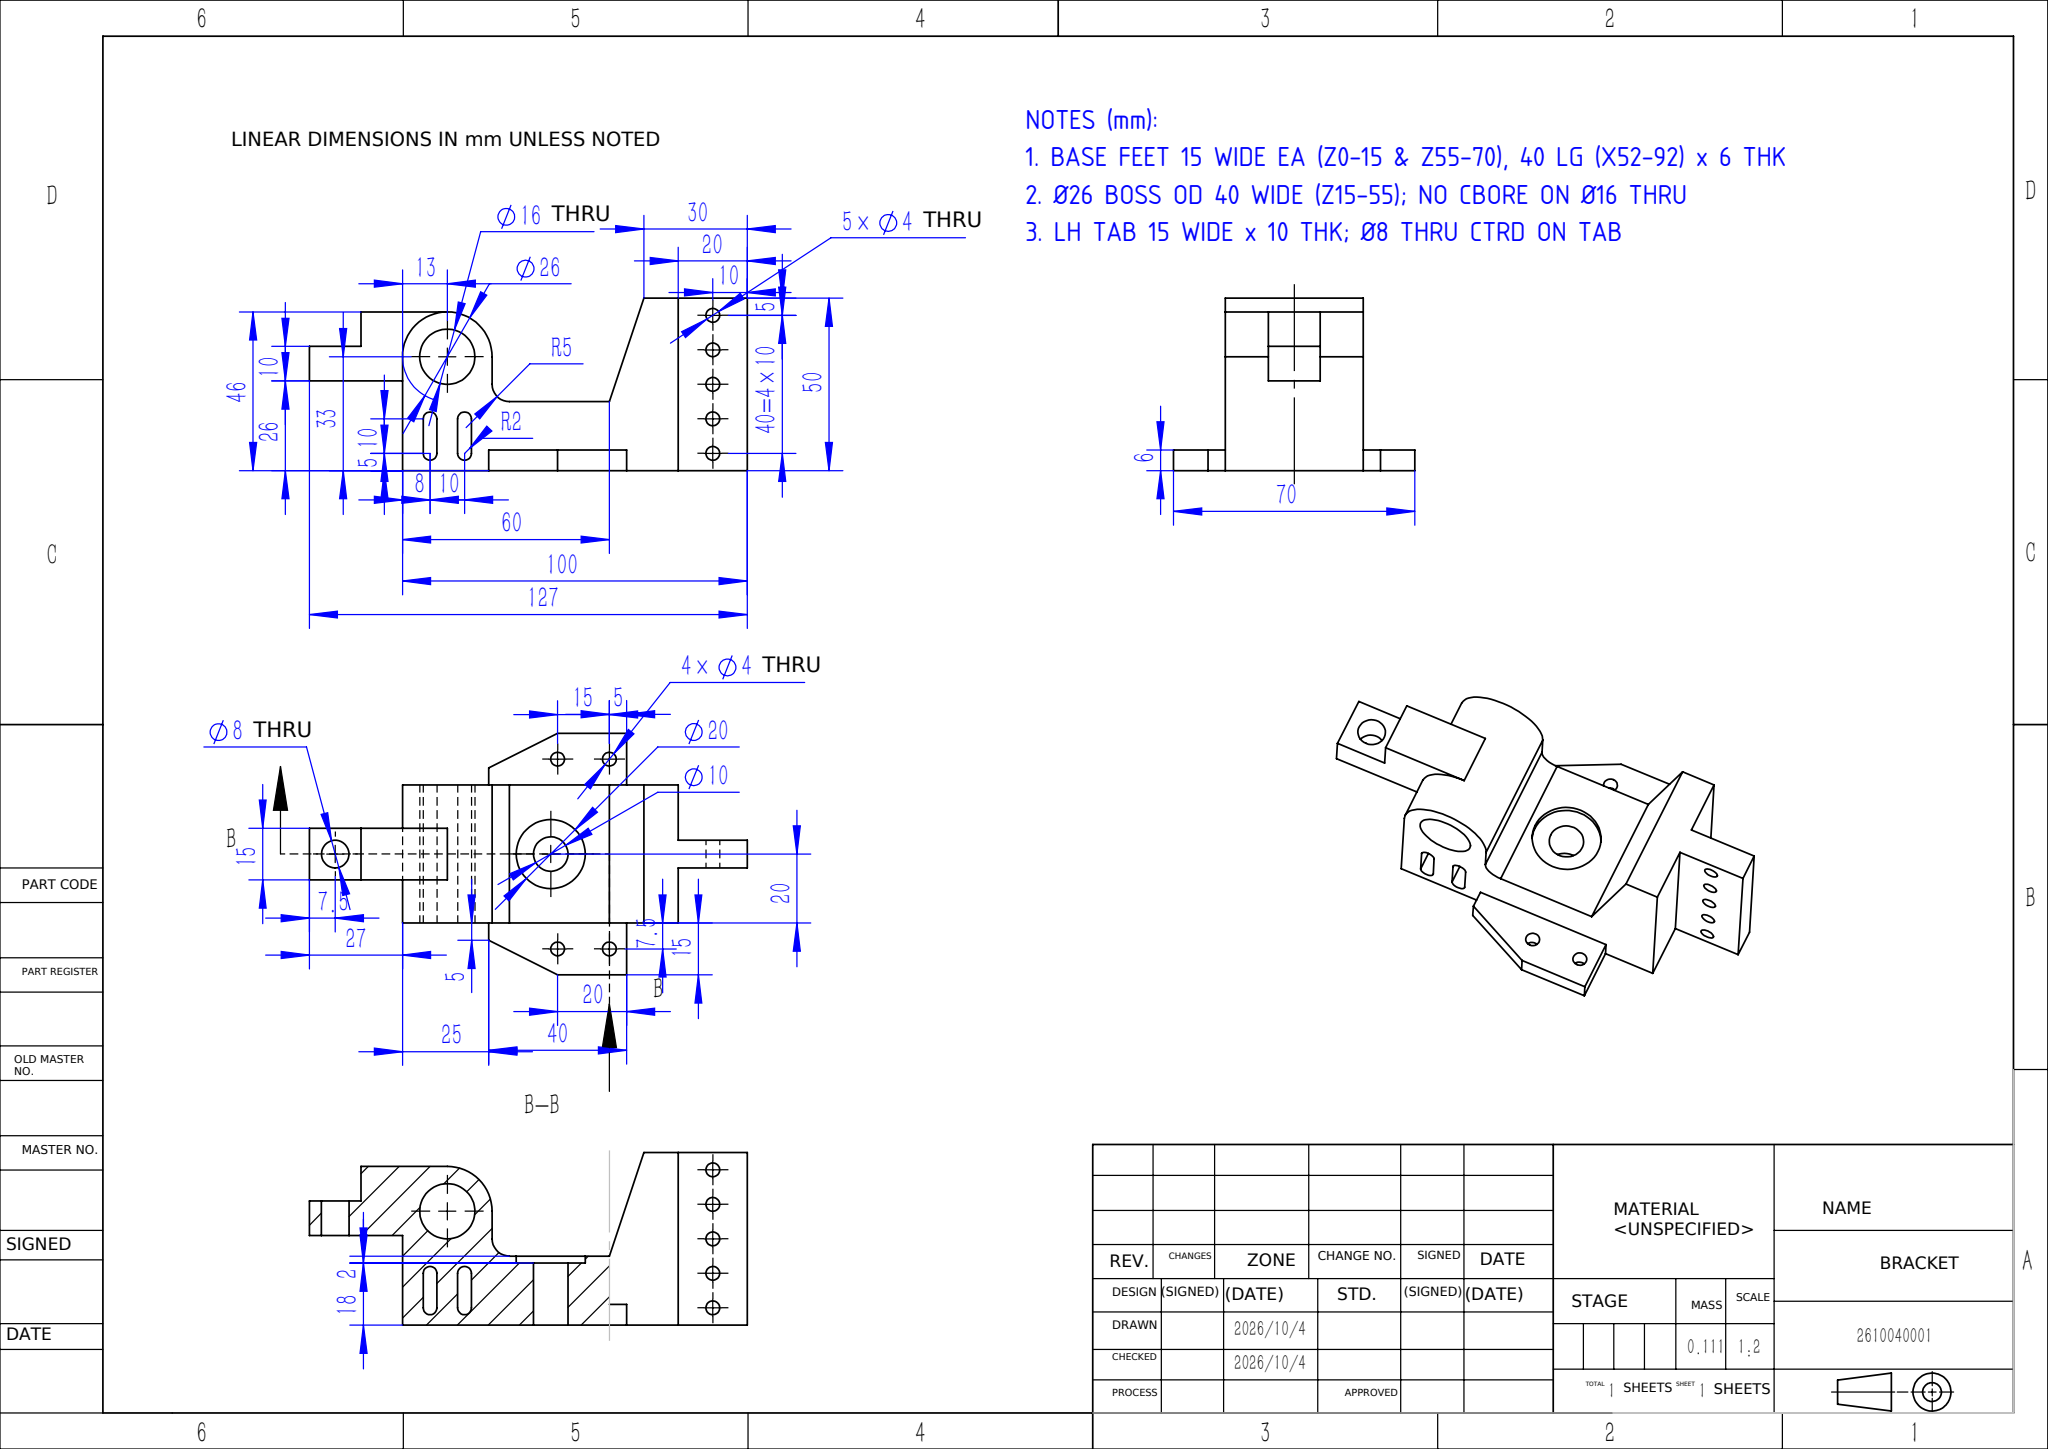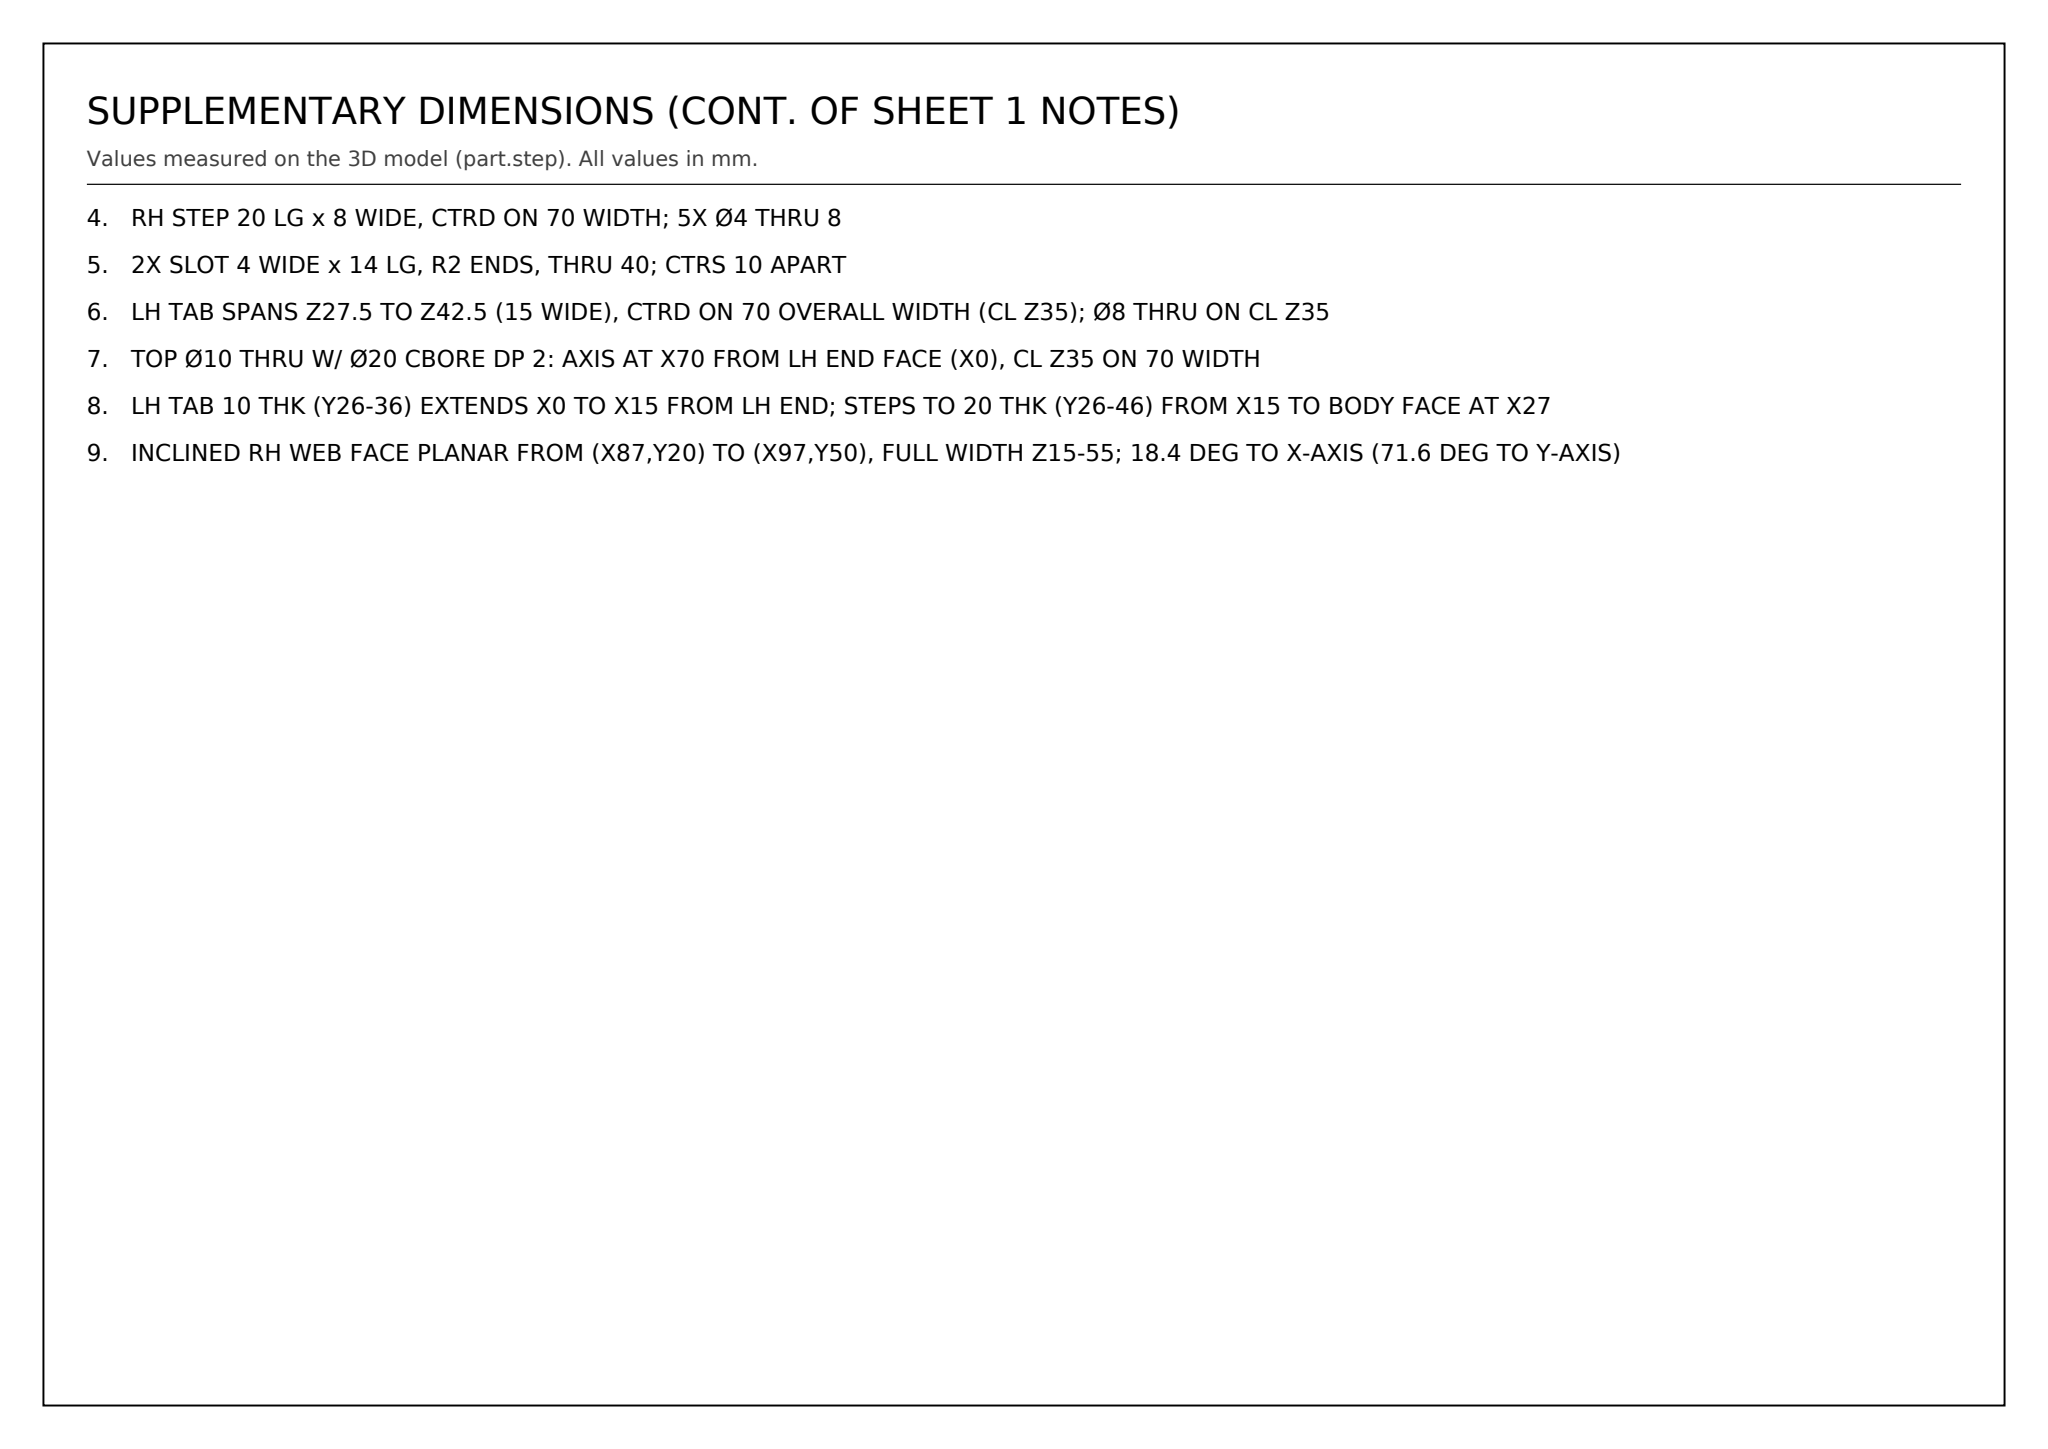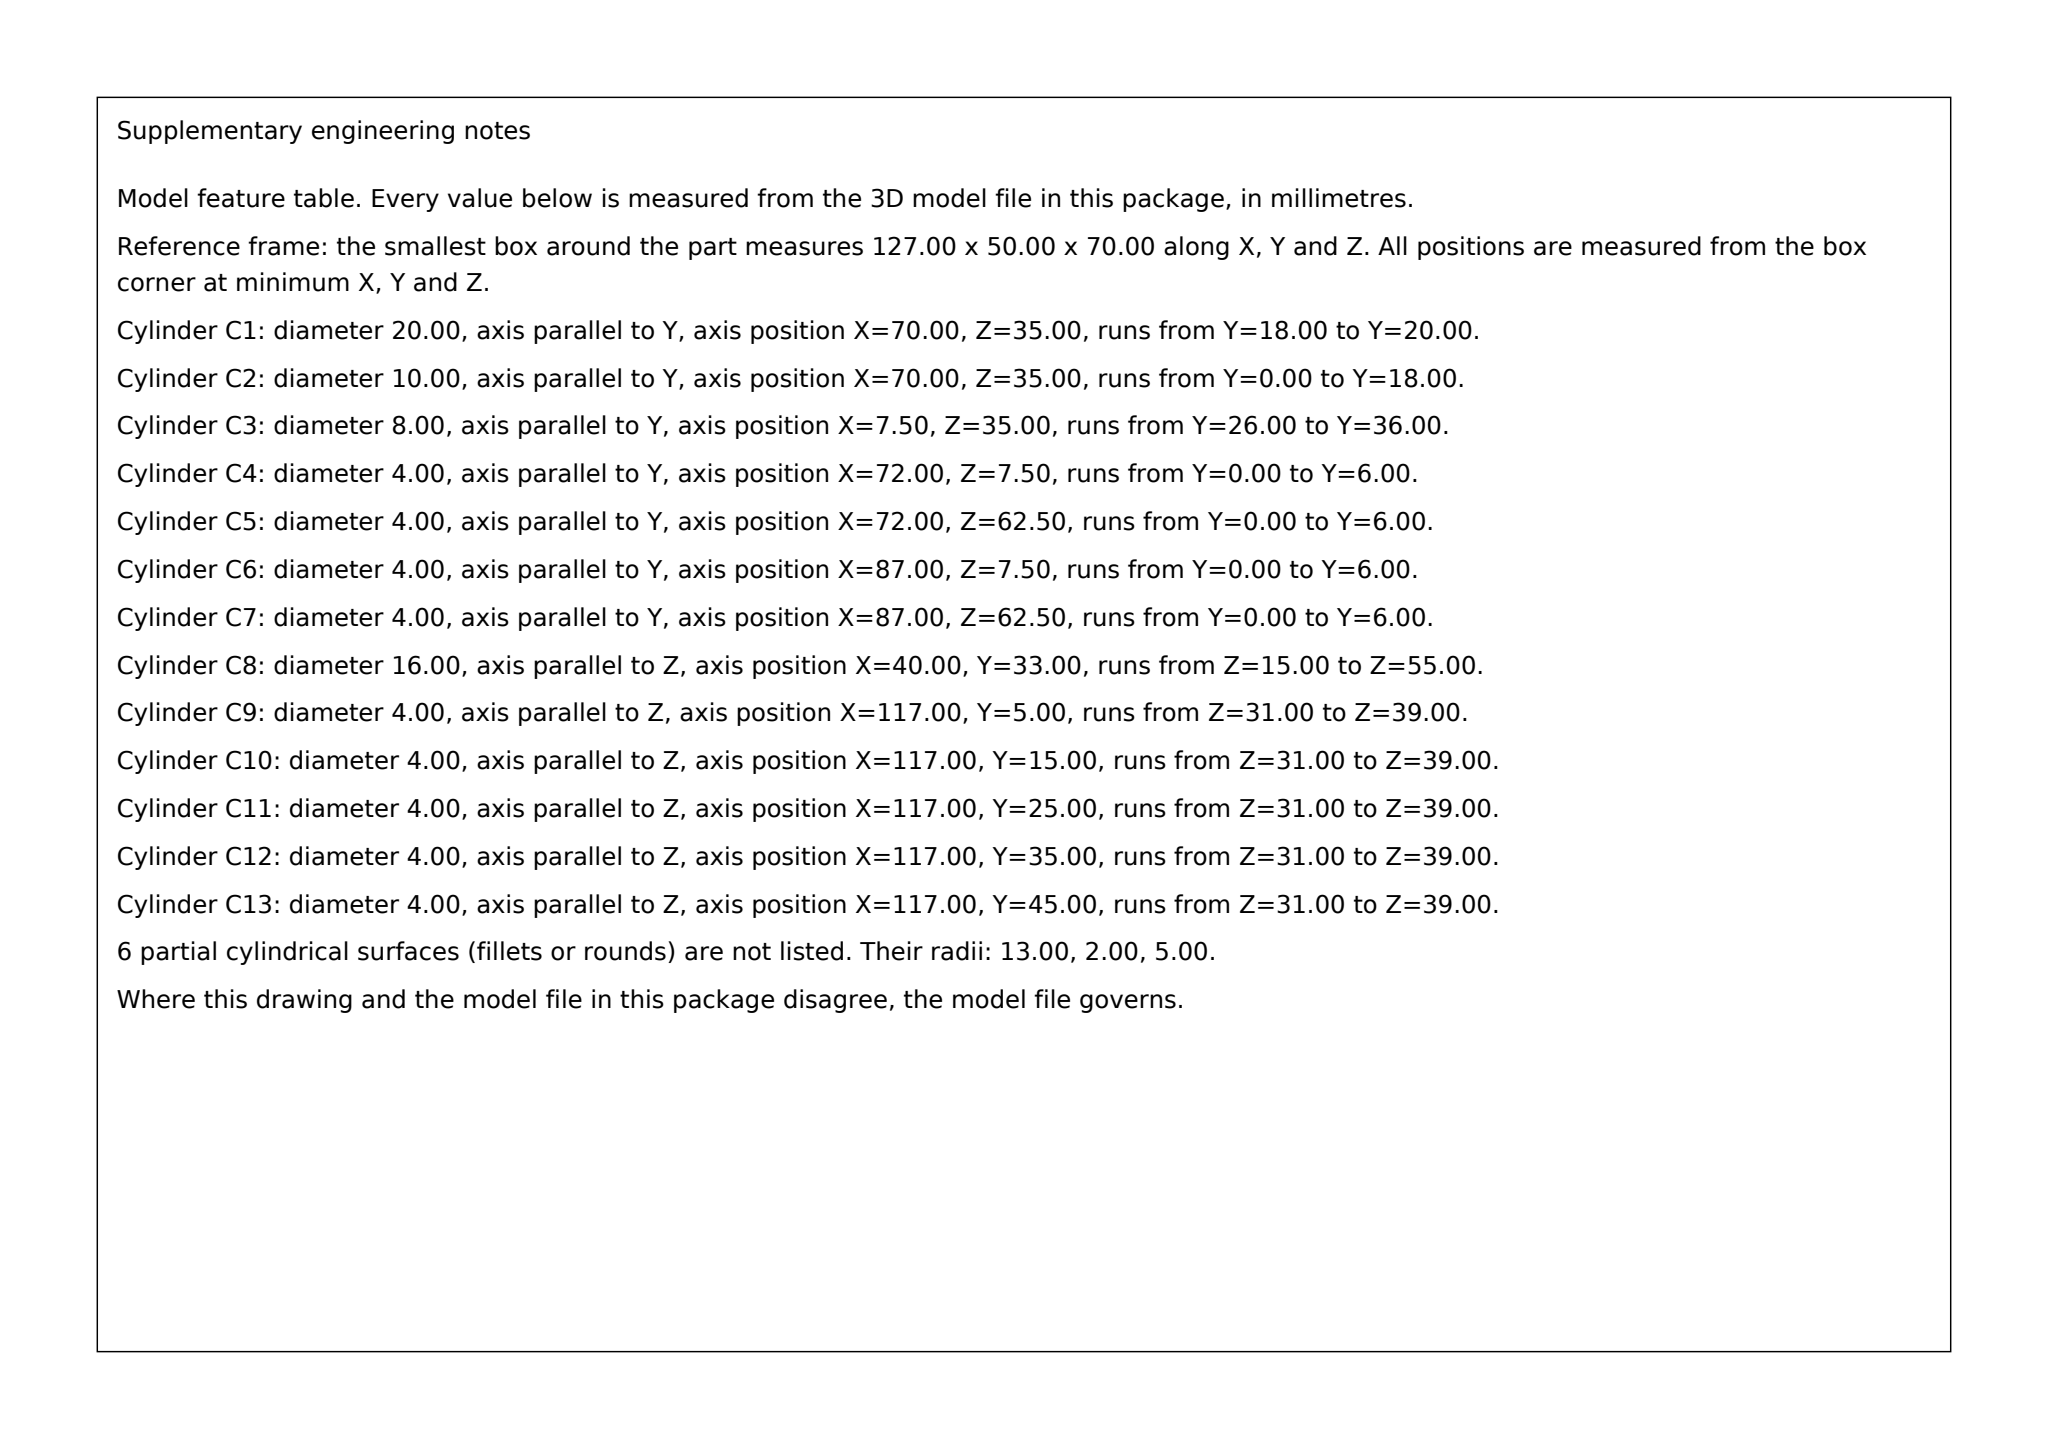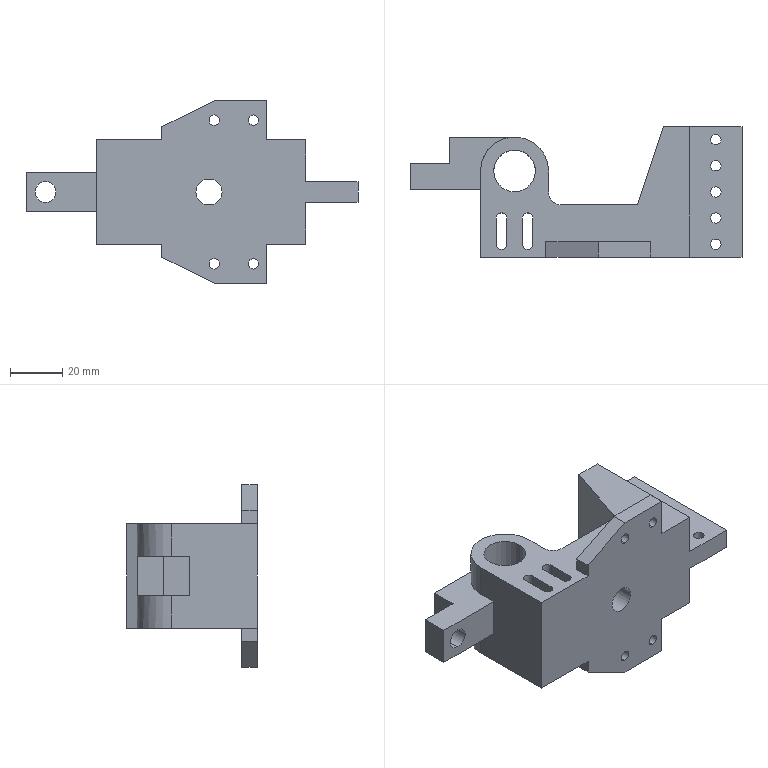Part | SolidWorks | mm | 1 solid | 67 faces | box 127 x 50 x 70 mm | volume 111150 mm3 | plane 35 | cylinder 32 | commonest cylinder face diameters 4 x22 10 x3 8 x2 20 x2 16 x2 26 x1
Drawing notes:
BASE FEET 15 WIDE EA (Z0-15 & Z55-70), 40 LG (X52-92) x 6 THK | from the solid: z-planes 0,15,55,70; x-planes 52 & 92; y-plane 6; dia4 axis y at z7.5 & z62.5 len 6
Ø26 BOSS OD 40 WIDE (Z15-55); NO CBORE ON Ø16 THRU | from the solid: Cyl Ø26 axis z at (40,33) len 40, z planes 15 & 55; Ø16 same axis len 40 thru, no intermediate z face
LH TAB 15 WIDE x 10 THK; Ø8 THRU CTRD ON TAB | from the solid: x-planes 0,15,27; z-planes 27.5/42.5; dia8 axis y at (7.5,35) len 10
RH STEP 20 LG x 8 WIDE, CTRD ON 70 WIDTH; 5X Ø4 THRU 8 | from the solid: x-planes 107 & 127; z-planes 31 & 39; 5X dia4 axis z at x117 len 8
2X SLOT 4 WIDE x 14 LG, R2 ENDS, THRU 40; CTRS 10 APART | from the solid: dia4 axis z at (35,5),(35,15),(45,5),(45,15) len 40 -> 4 wide, 14 OAL
LH TAB SPANS Z27.5 TO Z42.5 (15 WIDE), CTRD ON 70 OVERALL WIDTH (CL Z35); Ø8 THRU ON CL Z35 | from the solid: axis_planes x=0.0 extent z [27.5,42.5]; hole/bore dia 8.0 axis y at [7.5, null, 35.0] from 26.0 to 36.0
TOP Ø10 THRU W/ Ø20 CBORE DP 2: AXIS AT X70 FROM LH END FACE (X0), CL Z35 ON 70 WIDTH | from the solid: Ø10 bore, axis y at (x70, z35), from y0 to y18; Ø20 bore same axis from y18 to y20 (entry face y=20, cbore dp 2). The Ø10 reaches the bottom face y=0 (y=0 plane area 4231 only balances with the Ø10 opening), so the Ø10 is THRU the 20 thk section, not blind.
LH TAB 10 THK (Y26-36) EXTENDS X0 TO X15 FROM LH END; STEPS TO 20 THK (Y26-46) FROM X15 TO BODY FACE AT X27 | from the solid: axis_planes: y=36 over x[0,15] z[27.5,42.5]; y=46 over x[15,40] z[27.5,42.5]; x=15 over y[36,46]; x=27 over y[0,33]
INCLINED RH WEB FACE PLANAR FROM (X87,Y20) TO (X97,Y50), FULL WIDTH Z15-55; 18.4 DEG TO X-AXIS (71.6 DEG TO Y-AXIS) | from the solid: inclined_planes: angle_to_xyz_axes [18.4, 71.6, 90.0], bbox_from [87,20,15], size [10,30,40]
build123d program:
from build123d import *

# Parameters (mm, degrees)
BOSS_EXTRUDE1_DEPTH = 20
SKETCH2_W           = 20
SKETCH2_H           = 16
CUT_EXTRUDE1_DEPTH  = 114.578
SKETCH3_W           = 40
SKETCH3_H           = 15
BOSS_EXTRUDE2_DEPTH = 20
SKETCH4_W           = 15
SKETCH4_H           = 15
CUT_EXTRUDE2_DEPTH  = 10
BOSS_EXTRUDE3_DEPTH = 6
SKETCH6_R           = 8
CUT_EXTRUDE3_DEPTH  = 119.004
SKETCH7_R           = 10
CUT_EXTRUDE4_DEPTH  = 2
SKETCH8_R           = 5
CUT_EXTRUDE5_DEPTH  = 111.675
SKETCH9_R           = 2
CUT_EXTRUDE6_DEPTH  = 112.45
FILLET1_R           = 5
SKETCH10_R          = 4
CUT_EXTRUDE7_DEPTH  = 112.897
SKETCH11_R          = 2
CUT_EXTRUDE8_DEPTH  = 115.721
CUT_EXTRUDE9_DEPTH  = 119.004


with BuildPart() as part:
    # Sketch1 → Boss-Extrude1 (new, symmetric)
    with BuildSketch(Plane.XY):
        with BuildLine():
            Line((0, 0), (0, -20))
            Line((0, -20), (100, -20))
            Line((100, -20), (100, 30))
            Line((100, 30), (70, 30))
            Line((70, 30), (60, 0))
            Line((60, 0), (26, 0))
            Line((26, 0), (26, 13))
            ThreePointArc((26, 13), (13, 26), (0, 13))
            Line((0, 13), (0, 0))
        make_face()
    extrude(amount=BOSS_EXTRUDE1_DEPTH, both=True)

    # Sketch2 → Cut-Extrude1 (cut, through all)
    with BuildSketch(Plane(origin=(0, 30, 0), x_dir=(1, 0, 0), z_dir=(0, 1, 0))):
        with Locations((90, 12)):
            Rectangle(SKETCH2_W, SKETCH2_H)
        with Locations((90, -12)):
            Rectangle(SKETCH2_W, SKETCH2_H)
    extrude(amount=-CUT_EXTRUDE1_DEPTH, mode=Mode.SUBTRACT)

    # Sketch3 → Boss-Extrude2 (add)
    with BuildSketch(Plane(origin=(0, 26, 0), x_dir=(-1, 0, 0), z_dir=(0, -1, 0))):
        with Locations((7, 0)):
            Rectangle(SKETCH3_W, SKETCH3_H)
    extrude(amount=BOSS_EXTRUDE2_DEPTH)

    # Sketch4 → Cut-Extrude2 (cut)
    with BuildSketch(Plane(origin=(0, 26, 0), x_dir=(1, 0, 0), z_dir=(0, 1, 0))):
        with Locations((-19.5, 0)):
            Rectangle(SKETCH4_W, SKETCH4_H)
    extrude(amount=-CUT_EXTRUDE2_DEPTH, mode=Mode.SUBTRACT)

    # Sketch5 → Boss-Extrude3 (add)
    with BuildSketch(Plane.XZ.offset(20)):
        Polygon((65, 20), (65, 35), (45, 35), (25, 25), (25, 20), align=None)
        Polygon((25, -25), (25, -20), (65, -20), (65, -35), (45, -35), align=None)
    extrude(amount=-BOSS_EXTRUDE3_DEPTH)

    # Sketch6 → Cut-Extrude3 (cut, through all)
    with BuildSketch(Plane.XY.offset(20)):
        with Locations((13, 13)):
            Circle(SKETCH6_R)
    extrude(amount=-CUT_EXTRUDE3_DEPTH, mode=Mode.SUBTRACT)

    # Sketch7 → Cut-Extrude4 (cut)
    with BuildSketch(Plane(origin=(0, 0, 0), x_dir=(1, 0, 0), z_dir=(0, 1, 0))):
        with Locations(Location((43, 0, 0), (0, 0, 180))):
            Circle(SKETCH7_R)
    extrude(amount=-CUT_EXTRUDE4_DEPTH, mode=Mode.SUBTRACT)

    # Sketch8 → Cut-Extrude5 (cut, through all)
    with BuildSketch(Plane(origin=(0, -2, 0), x_dir=(1, 0, 0), z_dir=(0, 1, 0))):
        with Locations(Location((43, 0, 0), (0, 0, 180))):
            Circle(SKETCH8_R)
    extrude(amount=-CUT_EXTRUDE5_DEPTH, mode=Mode.SUBTRACT)

    # Sketch9 → Cut-Extrude6 (cut, through all)
    with BuildSketch(Plane.XY.offset(4)):
        with Locations((90, 25)):
            Circle(SKETCH9_R)
        with Locations((90, 15)):
            Circle(SKETCH9_R)
        with Locations((90, 5)):
            Circle(SKETCH9_R)
        with Locations((90, -5)):
            Circle(SKETCH9_R)
        with Locations((90, -15)):
            Circle(SKETCH9_R)
    extrude(amount=-CUT_EXTRUDE6_DEPTH, mode=Mode.SUBTRACT)

    # Fillet1
    fillet1_edges = [part.edges().sort_by_distance(p)[0] for p in [
        (26, 0, 0),
    ]]
    fillet(fillet1_edges, radius=FILLET1_R)

    # Sketch10 → Cut-Extrude7 (cut, through all)
    with BuildSketch(Plane(origin=(0, 16, 0), x_dir=(1, 0, 0), z_dir=(0, 1, 0))):
        with Locations(Location((-19.5, 0, 0), (0, 0, 270))):
            Circle(SKETCH10_R)
    extrude(amount=-CUT_EXTRUDE7_DEPTH, mode=Mode.SUBTRACT)

    # Sketch11 → Cut-Extrude8 (cut, through all)
    with BuildSketch(Plane(origin=(0, -14, 0), x_dir=(1, 0, 0), z_dir=(0, 1, 0))):
        with Locations(Location((60, -27.5, 0), (0, 0, 270))):
            Circle(SKETCH11_R)
        with Locations(Location((45, -27.5, 0), (0, 0, 270))):
            Circle(SKETCH11_R)
        with Locations(Location((60, 27.5, 0), (0, 0, 90))):
            Circle(SKETCH11_R)
        with Locations(Location((45, 27.5, 0), (0, 0, 90))):
            Circle(SKETCH11_R)
    extrude(amount=-CUT_EXTRUDE8_DEPTH, mode=Mode.SUBTRACT)

    # Sketch12 → Cut-Extrude9 (cut, through all)
    with BuildSketch(Plane.XY.offset(20)):
        with BuildLine():
            Line((10, -5), (10, -15))
            ThreePointArc((10, -15), (8, -17), (6, -15))
            Line((6, -15), (6, -5))
            ThreePointArc((6, -5), (8, -3), (10, -5))
        make_face()
        with BuildLine():
            Line((20, -5), (20, -15))
            ThreePointArc((20, -15), (18, -17), (16, -15))
            Line((16, -15), (16, -5))
            ThreePointArc((16, -5), (18, -3), (20, -5))
        make_face()
    extrude(amount=-CUT_EXTRUDE9_DEPTH, mode=Mode.SUBTRACT)


solid = part.part